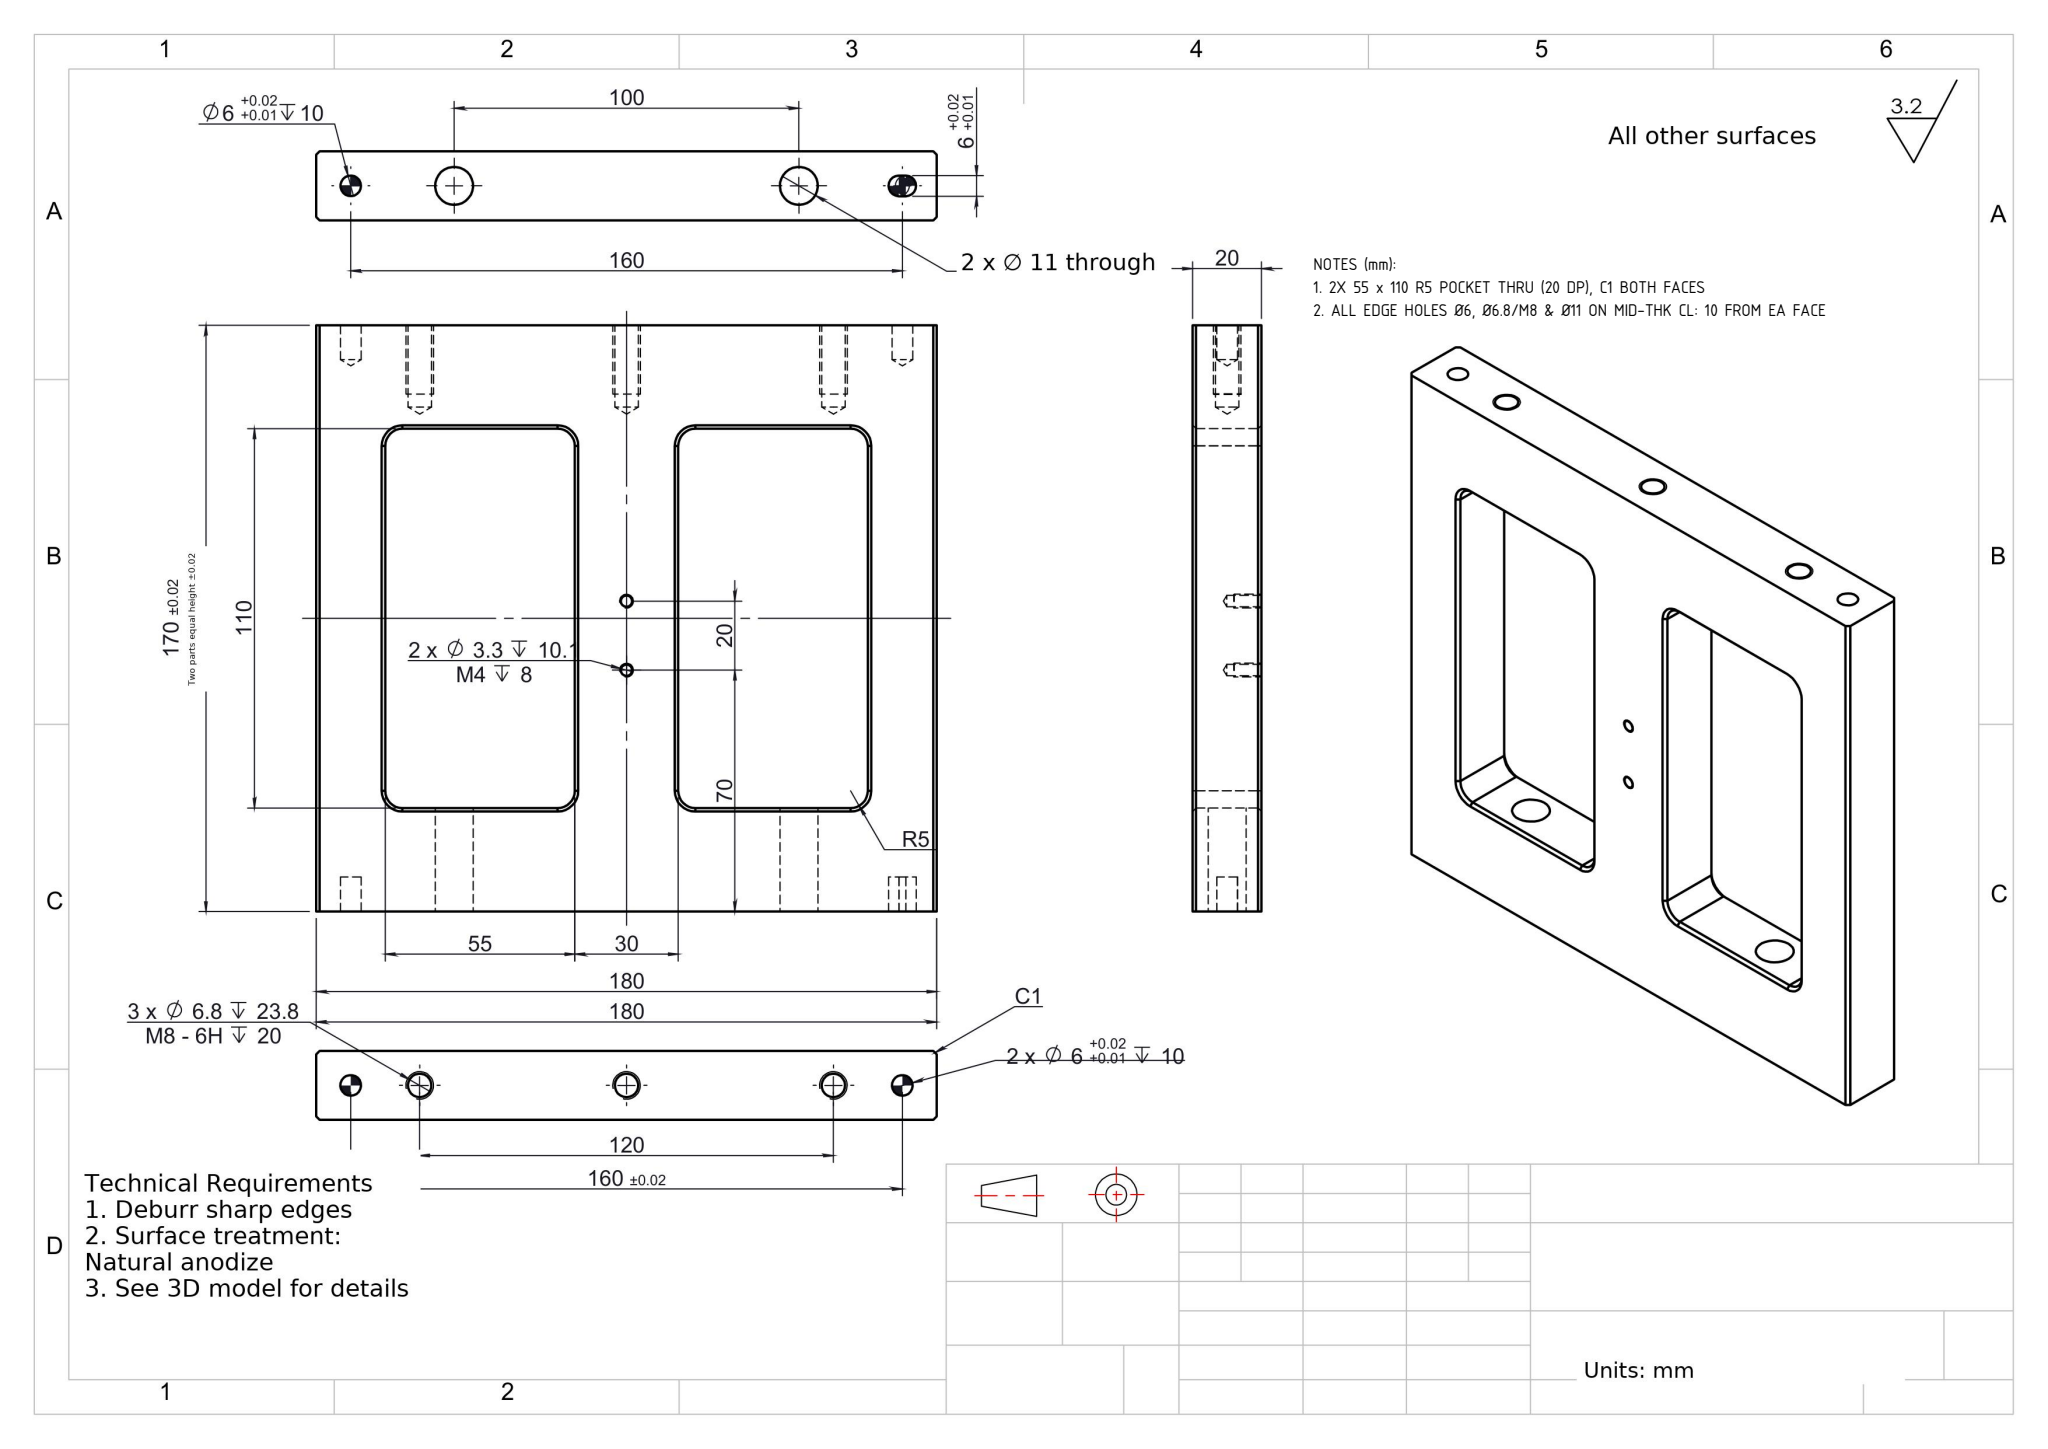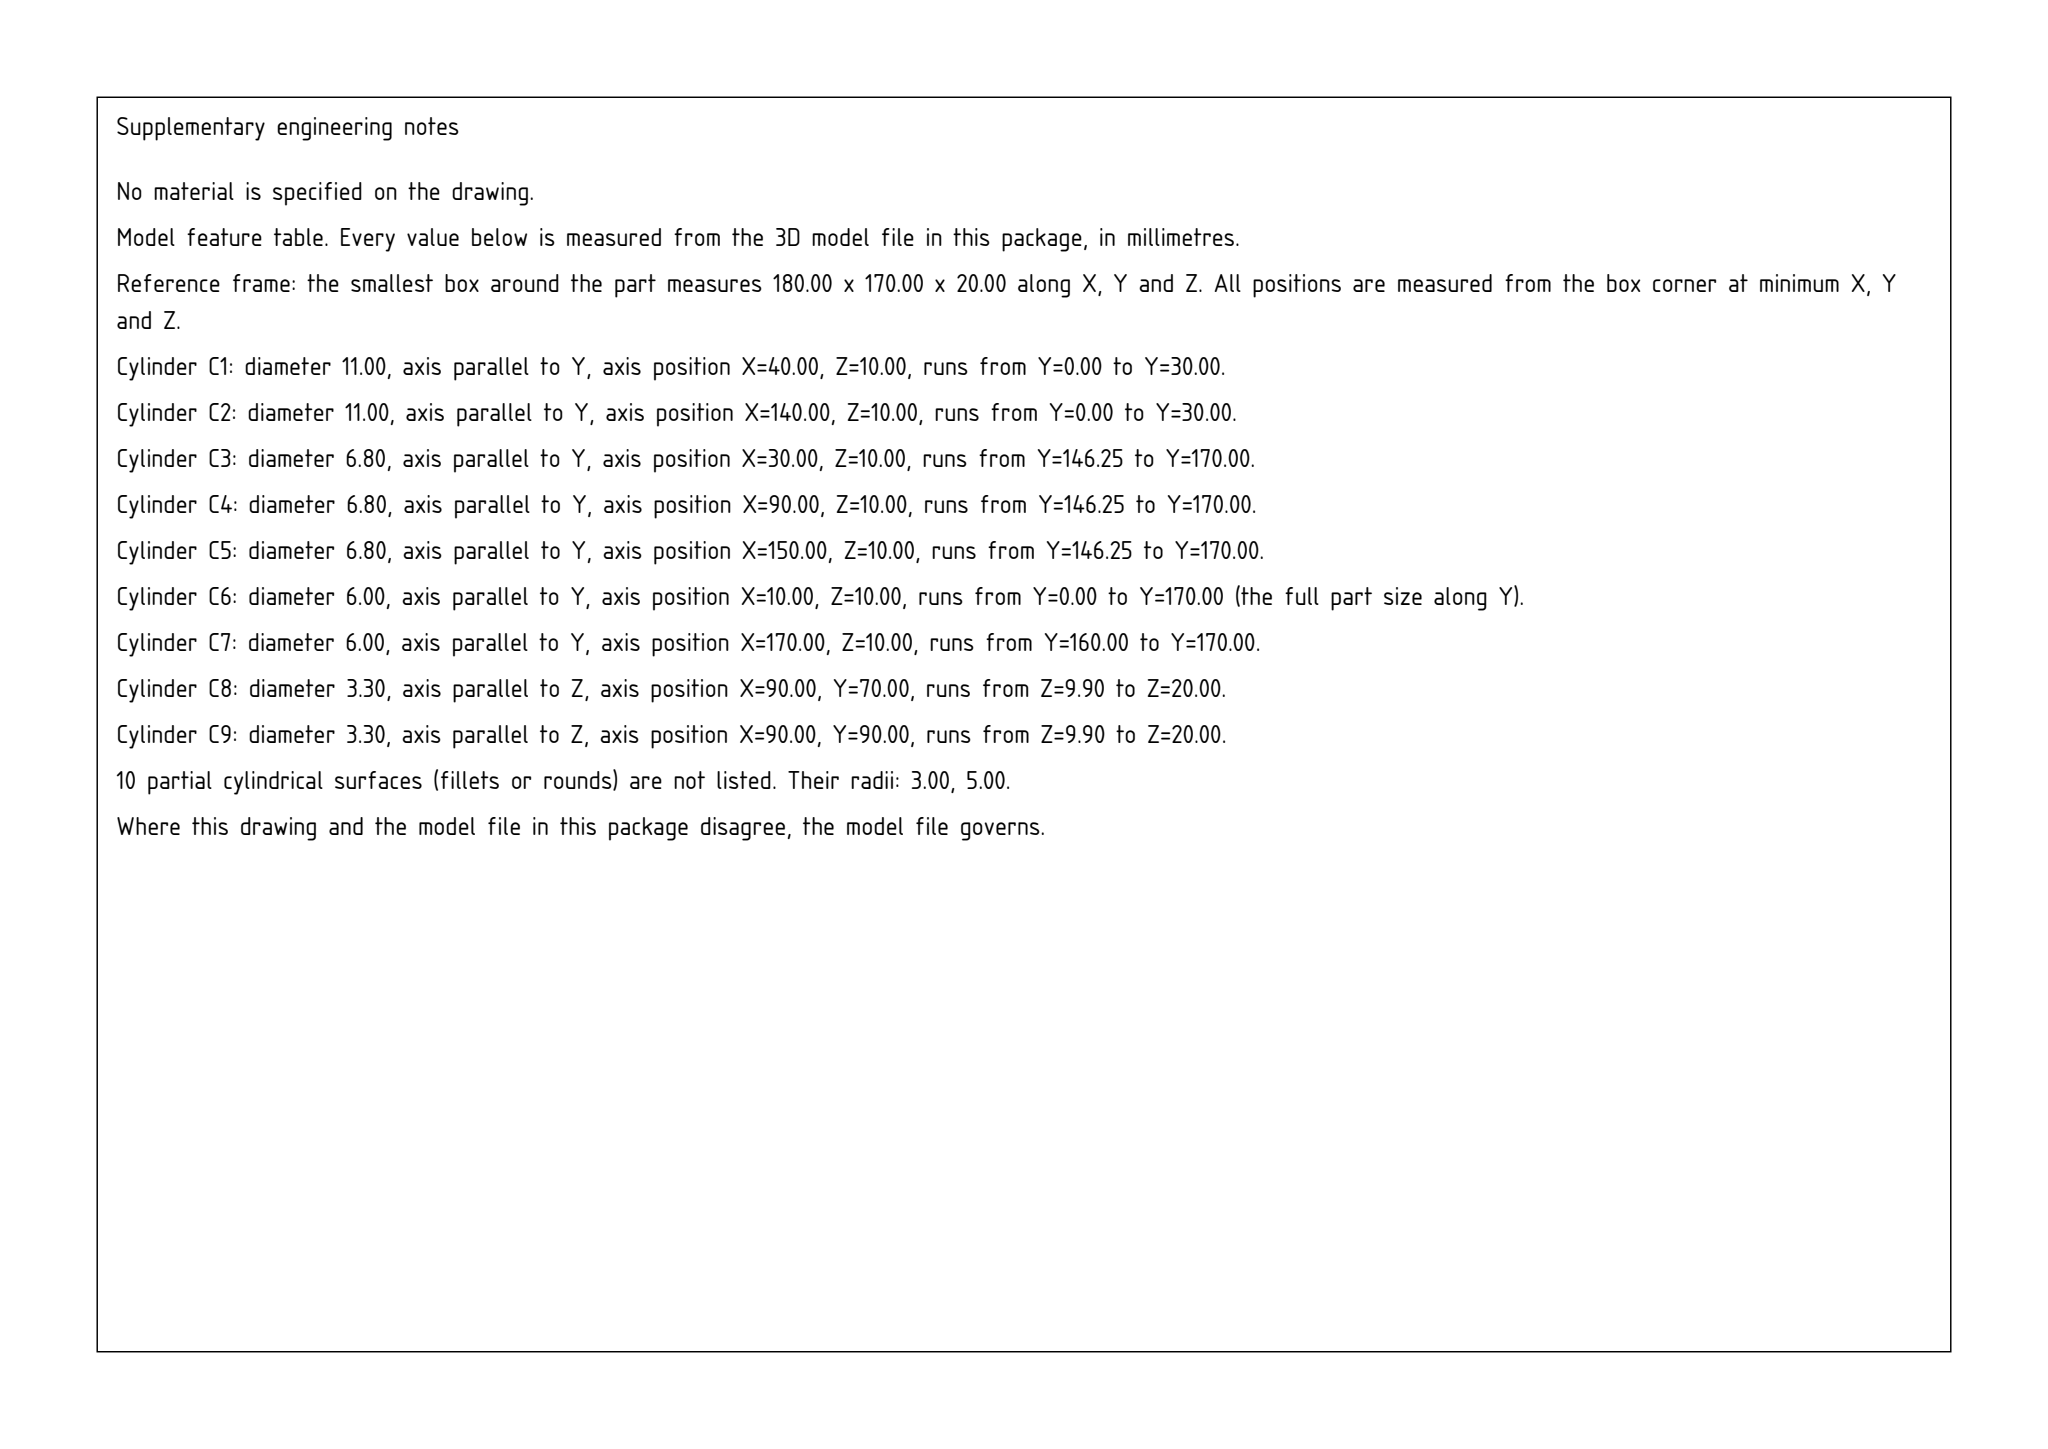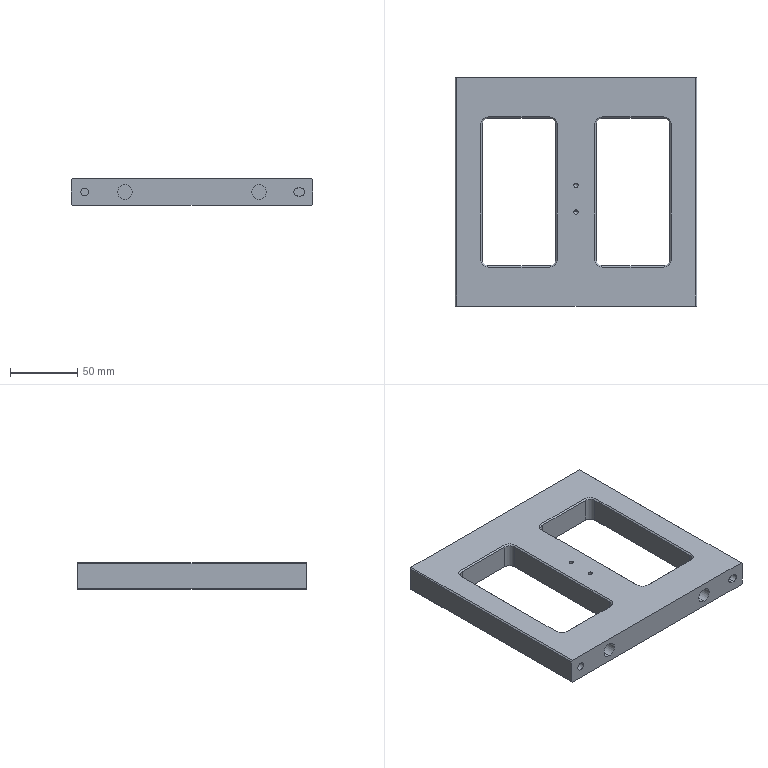Part | SolidWorks | mm | 1 solid | 99 faces | box 180 x 170 x 20 mm | volume 360044 mm3 | plane 38 | cylinder 31 | cone 30 | commonest cylinder face diameters 6 x9 10 x8 6.8 x6 3.3 x4 11 x4
Drawing notes:
2X 55 x 110 R5 POCKET THRU (20 DP), C1 BOTH FACES | from the solid: Pocket walls x=20/75 & 105/160, y=30/140; R5 corner cyls Ø10 len 18 + 1mm 90° chamfer each face = 20 = plate thk (bbox z=20); no floor plane in pockets
ALL EDGE HOLES Ø6, Ø6.8/M8 & Ø11 ON MID-THK CL: 10 FROM EA FACE | from the solid: Cylinders Ø6, Ø6.8 and Ø11, axis y, all at z=10.0 in 20.0 thk plate; Ø6.8 at x=30/90/150, Ø11 at x=40/140
build123d program:
from build123d import *

# Parameters (mm, degrees)
SKETCH1_W                     = 180
SKETCH1_H                     = 170
BOSS_EXTRUDE1_DEPTH           = 10
SIZE_MM_DOWEL_PIN_HOLE1_D     = 6
SIZE_MM_DOWEL_PIN_HOLE1_DEPTH = 10
SIZE_MM_DOWEL_PIN_HOLE1_TIP   = 1.803
SKETCH4_R                     = 3
CUT_EXTRUDE1_DEPTH            = 10
CUT_EXTRUDE2_DEPTH            = 126.399
M10_CLEARANCE_HOLE1_D         = 11
M10_CLEARANCE_HOLE1_DEPTH     = 30
M8_TAPPED_HOLE1_D             = 6.8
M8_TAPPED_HOLE1_DEPTH         = 23.75
M8_TAPPED_HOLE1_TIP           = 2.043
CHAMFER1_SIZE                 = 1
M4_TAPPED_HOLE1_D             = 3.3
M4_TAPPED_HOLE1_DEPTH         = 10.1
M4_TAPPED_HOLE1_TIP           = 0.9914


with BuildPart() as part:
    # Sketch1 → Boss-Extrude1 (new, symmetric)
    with BuildSketch(Plane.XY):
        Rectangle(SKETCH1_W, SKETCH1_H)
    extrude(amount=BOSS_EXTRUDE1_DEPTH, both=True)

    # Size mm Dowel Pin Hole1
    with Locations(Plane(origin=(0, 85, 0), x_dir=(1, 0, 0), z_dir=(0, 1, 0))):
        with Locations((-80, 0), (80, 0)):
            Hole(SIZE_MM_DOWEL_PIN_HOLE1_D / 2, depth=SIZE_MM_DOWEL_PIN_HOLE1_DEPTH)
            with Locations((0, 0, -(SIZE_MM_DOWEL_PIN_HOLE1_DEPTH + SIZE_MM_DOWEL_PIN_HOLE1_TIP / 2))):  # 118° drill point
                Cone(0, SIZE_MM_DOWEL_PIN_HOLE1_D / 2, SIZE_MM_DOWEL_PIN_HOLE1_TIP, mode=Mode.SUBTRACT)

    # Sketch4 → Cut-Extrude1 (cut)
    with BuildSketch(Plane.XZ.offset(85)):
        with Locations(Location((-80, 0, 0), (0, 0, 90))):
            Circle(SKETCH4_R)
        with BuildLine():
            Line((79, 3), (81, 3))
            ThreePointArc((81, 3), (84, 0), (81, -3))
            Line((81, -3), (79, -3))
            ThreePointArc((79, -3), (76, 0), (79, 3))
        make_face()
    extrude(amount=-CUT_EXTRUDE1_DEPTH, mode=Mode.SUBTRACT)

    # Sketch5 → Cut-Extrude2 (cut, through all)
    with BuildSketch(Plane.XY.offset(10)):
        with BuildLine():
            Line((-65, 55), (-20, 55))
            ThreePointArc((-20, 55), (-16.464, 53.536), (-15, 50))
            Line((-15, 50), (-15, -50))
            ThreePointArc((-15, -50), (-16.464, -53.536), (-20, -55))
            Line((-20, -55), (-65, -55))
            ThreePointArc((-65, -55), (-68.536, -53.536), (-70, -50))
            Line((-70, -50), (-70, 50))
            ThreePointArc((-70, 50), (-68.536, 53.536), (-65, 55))
        make_face()
        with BuildLine():
            Line((15, 50), (15, -50))
            ThreePointArc((15, -50), (16.464, -53.536), (20, -55))
            Line((20, -55), (65, -55))
            ThreePointArc((65, -55), (68.536, -53.536), (70, -50))
            Line((70, -50), (70, 50))
            ThreePointArc((70, 50), (68.536, 53.536), (65, 55))
            Line((65, 55), (20, 55))
            ThreePointArc((20, 55), (16.464, 53.536), (15, 50))
        make_face()
    extrude(amount=-CUT_EXTRUDE2_DEPTH, mode=Mode.SUBTRACT)

    # M10 Clearance Hole1
    with Locations(Plane(origin=(0, -85, 0), x_dir=(-1, 0, 0), z_dir=(0, -1, 0))):
        with Locations((50, 0), (-50, 0)):
            Hole(M10_CLEARANCE_HOLE1_D / 2, depth=M10_CLEARANCE_HOLE1_DEPTH)

    # M8 Tapped Hole1
    with Locations(Plane(origin=(0, 85, 0), x_dir=(1, 0, 0), z_dir=(0, 1, 0))):
        with Locations((-60, 0), (0, 0), (60, 0)):
            Hole(M8_TAPPED_HOLE1_D / 2, depth=M8_TAPPED_HOLE1_DEPTH)
            with Locations((0, 0, -(M8_TAPPED_HOLE1_DEPTH + M8_TAPPED_HOLE1_TIP / 2))):  # 118° drill point
                Cone(0, M8_TAPPED_HOLE1_D / 2, M8_TAPPED_HOLE1_TIP, mode=Mode.SUBTRACT)

    # Chamfer1
    chamfer1_edges = [part.edges().sort_by_distance(p)[0] for p in [
        (90, 0, 10),
        (-90, 0, 10),
        (-68.536, -53.536, -10),
        (90, 0, -10),
        (-70, 0, -10),
        (-68.536, 53.536, -10),
        (-42.5, 55, -10),
        (-16.464, 53.536, -10),
        (-15, 0, -10),
        (-16.464, -53.536, -10),
        (-42.5, -55, -10),
        (-68.536, -53.536, 10),
        (-42.5, -55, 10),
        (-16.464, -53.536, 10),
        (-15, 0, 10),
        (-16.464, 53.536, 10),
        (-42.5, 55, 10),
        (-68.536, 53.536, 10),
        (-70, 0, 10),
        (-90, 0, -10),
        (68.536, 53.536, -10),
        (70, 0, -10),
        (68.536, -53.536, -10),
        (42.5, -55, -10),
        (16.464, -53.536, -10),
        (15, 0, -10),
        (16.464, 53.536, -10),
        (42.5, 55, -10),
        (68.536, 53.536, 10),
        (42.5, 55, 10),
        (16.464, 53.536, 10),
        (15, 0, 10),
        (16.464, -53.536, 10),
        (42.5, -55, 10),
        (68.536, -53.536, 10),
        (70, 0, 10),
    ]]
    chamfer(chamfer1_edges, length=CHAMFER1_SIZE)

    # M4 Tapped Hole1
    with Locations(Plane.XY.offset(10)):
        with Locations((0, 5), (0, -15)):
            Hole(M4_TAPPED_HOLE1_D / 2, depth=M4_TAPPED_HOLE1_DEPTH)
            with Locations((0, 0, -(M4_TAPPED_HOLE1_DEPTH + M4_TAPPED_HOLE1_TIP / 2))):  # 118° drill point
                Cone(0, M4_TAPPED_HOLE1_D / 2, M4_TAPPED_HOLE1_TIP, mode=Mode.SUBTRACT)


solid = part.part